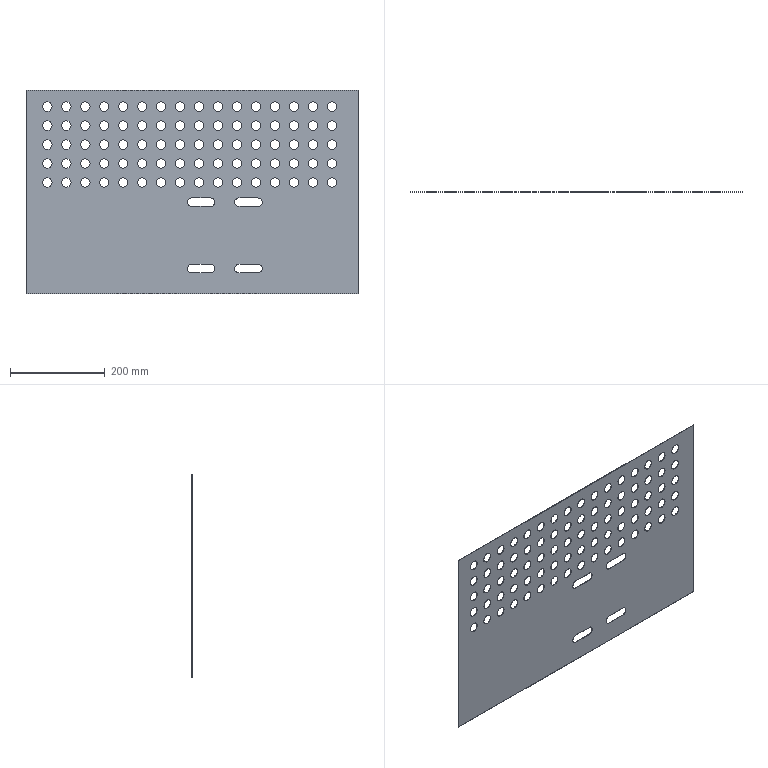Component | SolidWorks | CCQ-1.1-7BasePlate-1 | 1 solid | 186 faces | volume 271969 mm3 | cylinder 172 | plane 14 | commonest cylinder face diameters 20 x160 18 x12 | material 304